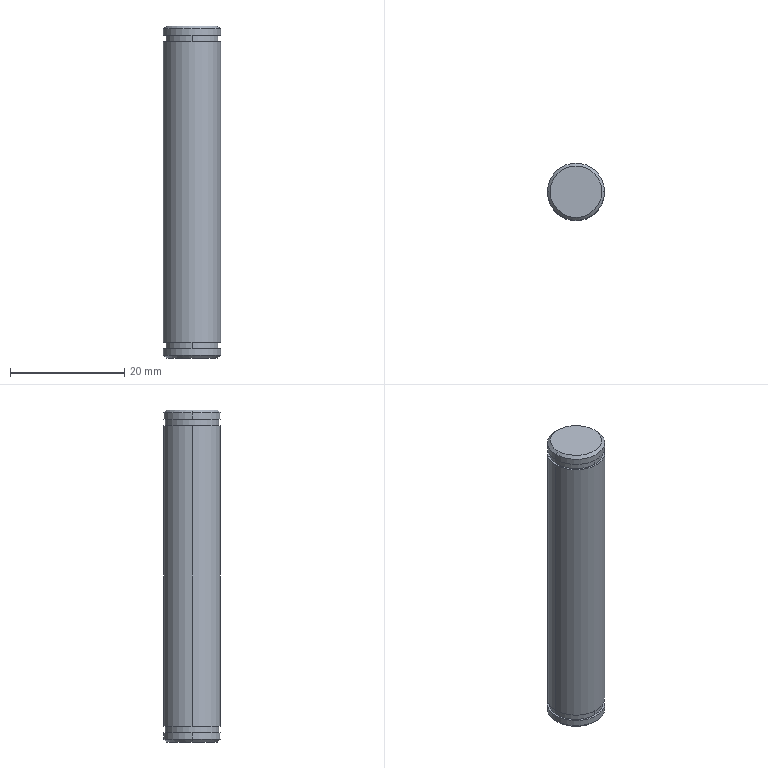Component | SolidWorks | 170423A4-IdlerAssembly5-10_170423A4-IdlerAxis1-1 | 1 solid | 20 faces | box 10 x 10 x 58 mm | volume 4523 mm3 | cylinder 10 | plane 6 | cone 4 | commonest cylinder face diameters 10 x6 9.3 x4
build123d program:
from build123d import *

# Parameters (mm, degrees)
SKETCH1_R           = 5
BOSS_EXTRUDE1_DEPTH = 58
SKETCH2_W           = 1.15
SKETCH2_H           = 0.35
CHAMFER1_SIZE       = 0.5


with BuildPart() as part:
    # Sketch1 → Boss-Extrude1 (new body)
    with BuildSketch(Plane.XY):
        with Locations(Location((0, 0, 0), (0, 0, 180))):
            Circle(SKETCH1_R)
    extrude(amount=BOSS_EXTRUDE1_DEPTH)

    # Sketch2 → Cut-Revolve1 (revolve, cut)
    with BuildSketch(Plane(origin=(0, 0, 0), x_dir=(0, 0, -1), z_dir=(1, 0, 0)), mode=Mode.PRIVATE) as cut_revolve1_sk:
        with Locations((-55.825, 4.825)):
            Rectangle(SKETCH2_W, SKETCH2_H)
        with Locations((-2.175, 4.825)):
            Rectangle(SKETCH2_W, SKETCH2_H)
    revolve(cut_revolve1_sk.sketch.rotate(Axis((0, 0, 58), (0, 0, -1)), 180), axis=Axis((0, 0, 58), (0, 0, -1)), mode=Mode.SUBTRACT)

    # Chamfer1
    chamfer1_edges = [part.edges().sort_by_distance(p)[0] for p in [
        (5, 0, 0),
        (5, 0, 58),
    ]]
    chamfer(chamfer1_edges, length=CHAMFER1_SIZE)


solid = part.part

# Placed as in the assembly
solid = solid.moved(Location((-162.746, 8.712, 412), (0, 0, 0)))
STEP:
#1=COLOUR_RGB('',0.7922,0.8196,0.9333);
#2=FILL_AREA_STYLE_COLOUR('',#1);
#3=FILL_AREA_STYLE('',(#2));
#4=SURFACE_STYLE_FILL_AREA(#3);
#5=SURFACE_SIDE_STYLE('',(#4));
#6=SURFACE_STYLE_USAGE(.BOTH.,#5);
#7=PRESENTATION_STYLE_ASSIGNMENT((#6));
#8=CARTESIAN_POINT('',(-6.585,0.343,18.504));
#9=VERTEX_POINT('',#8);
#10=CARTESIAN_POINT('',(-6.23,0.343,18.504));
#11=VERTEX_POINT('',#10);
#12=CARTESIAN_POINT('',(-6.407,0.343,18.504));
#13=DIRECTION('',(0.,0.,1.));
#14=DIRECTION('',(-1.,0.,0.));
#15=AXIS2_PLACEMENT_3D('',#12,#13,#14);
#16=CIRCLE('',#15,0.1772);
#17=EDGE_CURVE('',#9,#11,#16,.T.);
#18=ORIENTED_EDGE('',*,*,#17,.F.);
#19=CARTESIAN_POINT('',(-6.604,0.343,18.484));
#20=VERTEX_POINT('',#19);
#21=CARTESIAN_POINT('',(-6.585,0.343,18.504));
#22=DIRECTION('',(-0.7071,-0.,-0.7071));
#23=VECTOR('',#22,39.37);
#24=LINE('',#21,#23);
#25=EDGE_CURVE('',#9,#20,#24,.T.);
#26=ORIENTED_EDGE('',*,*,#25,.T.);
#27=CARTESIAN_POINT('',(-6.21,0.343,18.484));
#28=VERTEX_POINT('',#27);
#29=CARTESIAN_POINT('',(-6.407,0.343,18.484));
#30=DIRECTION('',(0.,0.,-1.));
#31=DIRECTION('',(-1.,0.,0.));
#32=AXIS2_PLACEMENT_3D('',#29,#30,#31);
#33=CIRCLE('',#32,0.1969);
#34=EDGE_CURVE('',#28,#20,#33,.T.);
#35=ORIENTED_EDGE('',*,*,#34,.F.);
#36=CARTESIAN_POINT('',(-6.23,0.343,18.504));
#37=DIRECTION('',(0.7071,0.,-0.7071));
#38=VECTOR('',#37,39.37);
#39=LINE('',#36,#38);
#40=EDGE_CURVE('',#11,#28,#39,.T.);
#41=ORIENTED_EDGE('',*,*,#40,.F.);
#42=EDGE_LOOP('',(#18,#26,#35,#41));
#43=FACE_OUTER_BOUND('',#42,.T.);
#44=CARTESIAN_POINT('',(-6.407,0.343,18.504));
#45=DIRECTION('',(0.,0.,-1.));
#46=DIRECTION('',(1.,0.,0.));
#47=AXIS2_PLACEMENT_3D('',#44,#45,#46);
#48=CONICAL_SURFACE('',#47,0.1772,0.7854);
#49=ADVANCED_FACE('',(#43),#48,.T.);
#50=CARTESIAN_POINT('',(-6.23,0.343,16.22));
#51=VERTEX_POINT('',#50);
#52=CARTESIAN_POINT('',(-6.585,0.343,16.22));
#53=VERTEX_POINT('',#52);
#54=CARTESIAN_POINT('',(-6.407,0.343,16.22));
#55=DIRECTION('',(0.,0.,-1.));
#56=DIRECTION('',(-1.,0.,0.));
#57=AXIS2_PLACEMENT_3D('',#54,#55,#56);
#58=CIRCLE('',#57,0.1772);
#59=EDGE_CURVE('',#51,#53,#58,.T.);
#60=ORIENTED_EDGE('',*,*,#59,.F.);
#61=CARTESIAN_POINT('',(-6.21,0.343,16.24));
#62=VERTEX_POINT('',#61);
#63=CARTESIAN_POINT('',(-6.21,0.343,16.24));
#64=DIRECTION('',(0.7071,-0.,0.7071));
#65=VECTOR('',#64,39.37);
#66=LINE('',#63,#65);
#67=EDGE_CURVE('',#51,#62,#66,.T.);
#68=ORIENTED_EDGE('',*,*,#67,.T.);
#69=CARTESIAN_POINT('',(-6.604,0.343,16.24));
#70=VERTEX_POINT('',#69);
#71=CARTESIAN_POINT('',(-6.407,0.343,16.24));
#72=DIRECTION('',(0.,0.,1.));
#73=DIRECTION('',(-1.,0.,0.));
#74=AXIS2_PLACEMENT_3D('',#71,#72,#73);
#75=CIRCLE('',#74,0.1969);
#76=EDGE_CURVE('',#70,#62,#75,.T.);
#77=ORIENTED_EDGE('',*,*,#76,.F.);
#78=CARTESIAN_POINT('',(-6.604,0.343,16.24));
#79=DIRECTION('',(-0.7071,-0.,0.7071));
#80=VECTOR('',#79,39.37);
#81=LINE('',#78,#80);
#82=EDGE_CURVE('',#53,#70,#81,.T.);
#83=ORIENTED_EDGE('',*,*,#82,.F.);
#84=EDGE_LOOP('',(#60,#68,#77,#83));
#85=FACE_OUTER_BOUND('',#84,.T.);
#86=CARTESIAN_POINT('',(-6.407,0.343,16.24));
#87=DIRECTION('',(0.,0.,1.));
#88=DIRECTION('',(-1.,0.,0.));
#89=AXIS2_PLACEMENT_3D('',#86,#87,#88);
#90=CONICAL_SURFACE('',#89,0.1969,0.7854);
#91=ADVANCED_FACE('',(#85),#90,.T.);
#92=CARTESIAN_POINT('',(-6.604,0.343,16.283));
#93=VERTEX_POINT('',#92);
#94=CARTESIAN_POINT('',(-6.21,0.343,16.283));
#95=VERTEX_POINT('',#94);
#96=CARTESIAN_POINT('',(-6.407,0.343,16.283));
#97=DIRECTION('',(-0.,0.,1.));
#98=DIRECTION('',(0.,1.,0.));
#99=AXIS2_PLACEMENT_3D('',#96,#97,#98);
#100=CIRCLE('',#99,0.1969);
#101=EDGE_CURVE('',#93,#95,#100,.T.);
#102=ORIENTED_EDGE('',*,*,#101,.F.);
#103=CARTESIAN_POINT('',(-6.604,0.343,18.504));
#104=DIRECTION('',(0.,0.,-1.));
#105=VECTOR('',#104,39.37);
#106=LINE('',#103,#105);
#107=EDGE_CURVE('',#93,#70,#106,.T.);
#108=ORIENTED_EDGE('',*,*,#107,.T.);
#109=ORIENTED_EDGE('',*,*,#76,.T.);
#110=CARTESIAN_POINT('',(-6.21,0.343,18.504));
#111=DIRECTION('',(0.,0.,-1.));
#112=VECTOR('',#111,39.37);
#113=LINE('',#110,#112);
#114=EDGE_CURVE('',#95,#62,#113,.T.);
#115=ORIENTED_EDGE('',*,*,#114,.F.);
#116=EDGE_LOOP('',(#102,#108,#109,#115));
#117=FACE_OUTER_BOUND('',#116,.T.);
#118=CARTESIAN_POINT('',(-6.407,0.343,18.504));
#119=DIRECTION('',(0.,0.,-1.));
#120=DIRECTION('',(1.,0.,0.));
#121=AXIS2_PLACEMENT_3D('',#118,#119,#120);
#122=CYLINDRICAL_SURFACE('',#121,0.1969);
#123=ADVANCED_FACE('',(#117),#122,.T.);
#124=CARTESIAN_POINT('',(-6.407,0.5261,16.283));
#125=VERTEX_POINT('',#124);
#126=CARTESIAN_POINT('',(-6.407,0.1599,16.283));
#127=VERTEX_POINT('',#126);
#128=CARTESIAN_POINT('',(-6.407,0.343,16.283));
#129=DIRECTION('',(-0.,0.,1.));
#130=DIRECTION('',(0.,1.,0.));
#131=AXIS2_PLACEMENT_3D('',#128,#129,#130);
#132=CIRCLE('',#131,0.1831);
#133=EDGE_CURVE('',#125,#127,#132,.T.);
#134=ORIENTED_EDGE('',*,*,#133,.T.);
#135=CARTESIAN_POINT('',(-6.407,0.1599,16.329));
#136=VERTEX_POINT('',#135);
#137=CARTESIAN_POINT('',(-6.407,0.1599,18.504));
#138=DIRECTION('',(-0.,0.,1.));
#139=VECTOR('',#138,39.37);
#140=LINE('',#137,#139);
#141=EDGE_CURVE('',#127,#136,#140,.T.);
#142=ORIENTED_EDGE('',*,*,#141,.T.);
#143=CARTESIAN_POINT('',(-6.407,0.5261,16.329));
#144=VERTEX_POINT('',#143);
#145=CARTESIAN_POINT('',(-6.407,0.343,16.329));
#146=DIRECTION('',(-0.,0.,1.));
#147=DIRECTION('',(0.,1.,0.));
#148=AXIS2_PLACEMENT_3D('',#145,#146,#147);
#149=CIRCLE('',#148,0.1831);
#150=EDGE_CURVE('',#144,#136,#149,.T.);
#151=ORIENTED_EDGE('',*,*,#150,.F.);
#152=CARTESIAN_POINT('',(-6.407,0.5261,18.504));
#153=DIRECTION('',(-0.,0.,1.));
#154=VECTOR('',#153,39.37);
#155=LINE('',#152,#154);
#156=EDGE_CURVE('',#125,#144,#155,.T.);
#157=ORIENTED_EDGE('',*,*,#156,.F.);
#158=EDGE_LOOP('',(#134,#142,#151,#157));
#159=FACE_OUTER_BOUND('',#158,.T.);
#160=CARTESIAN_POINT('',(-6.407,0.343,18.504));
#161=DIRECTION('',(-0.,0.,1.));
#162=DIRECTION('',(0.,1.,0.));
#163=AXIS2_PLACEMENT_3D('',#160,#161,#162);
#164=CYLINDRICAL_SURFACE('',#163,0.1831);
#165=ADVANCED_FACE('',(#159),#164,.T.);
#166=CARTESIAN_POINT('',(-6.407,0.5261,18.396));
#167=VERTEX_POINT('',#166);
#168=CARTESIAN_POINT('',(-6.407,0.1599,18.396));
#169=VERTEX_POINT('',#168);
#170=CARTESIAN_POINT('',(-6.407,0.343,18.396));
#171=DIRECTION('',(-0.,0.,1.));
#172=DIRECTION('',(0.,1.,0.));
#173=AXIS2_PLACEMENT_3D('',#170,#171,#172);
#174=CIRCLE('',#173,0.1831);
#175=EDGE_CURVE('',#167,#169,#174,.T.);
#176=ORIENTED_EDGE('',*,*,#175,.T.);
#177=CARTESIAN_POINT('',(-6.407,0.1599,18.441));
#178=VERTEX_POINT('',#177);
#179=CARTESIAN_POINT('',(-6.407,0.1599,18.504));
#180=DIRECTION('',(-0.,0.,1.));
#181=VECTOR('',#180,39.37);
#182=LINE('',#179,#181);
#183=EDGE_CURVE('',#169,#178,#182,.T.);
#184=ORIENTED_EDGE('',*,*,#183,.T.);
#185=CARTESIAN_POINT('',(-6.407,0.5261,18.441));
#186=VERTEX_POINT('',#185);
#187=CARTESIAN_POINT('',(-6.407,0.343,18.441));
#188=DIRECTION('',(-0.,0.,1.));
#189=DIRECTION('',(0.,1.,0.));
#190=AXIS2_PLACEMENT_3D('',#187,#188,#189);
#191=CIRCLE('',#190,0.1831);
#192=EDGE_CURVE('',#186,#178,#191,.T.);
#193=ORIENTED_EDGE('',*,*,#192,.F.);
#194=CARTESIAN_POINT('',(-6.407,0.5261,18.504));
#195=DIRECTION('',(-0.,0.,1.));
#196=VECTOR('',#195,39.37);
#197=LINE('',#194,#196);
#198=EDGE_CURVE('',#167,#186,#197,.T.);
#199=ORIENTED_EDGE('',*,*,#198,.F.);
#200=EDGE_LOOP('',(#176,#184,#193,#199));
#201=FACE_OUTER_BOUND('',#200,.T.);
#202=CARTESIAN_POINT('',(-6.407,0.343,18.504));
#203=DIRECTION('',(-0.,0.,1.));
#204=DIRECTION('',(0.,1.,0.));
#205=AXIS2_PLACEMENT_3D('',#202,#203,#204);
#206=CYLINDRICAL_SURFACE('',#205,0.1831);
#207=ADVANCED_FACE('',(#201),#206,.T.);
#208=ORIENTED_EDGE('',*,*,#34,.T.);
#209=CARTESIAN_POINT('',(-6.604,0.343,18.441));
#210=VERTEX_POINT('',#209);
#211=CARTESIAN_POINT('',(-6.604,0.343,18.504));
#212=DIRECTION('',(0.,0.,-1.));
#213=VECTOR('',#212,39.37);
#214=LINE('',#211,#213);
#215=EDGE_CURVE('',#20,#210,#214,.T.);
#216=ORIENTED_EDGE('',*,*,#215,.T.);
#217=CARTESIAN_POINT('',(-6.21,0.343,18.441));
#218=VERTEX_POINT('',#217);
#219=CARTESIAN_POINT('',(-6.407,0.343,18.441));
#220=DIRECTION('',(-0.,0.,1.));
#221=DIRECTION('',(0.,1.,0.));
#222=AXIS2_PLACEMENT_3D('',#219,#220,#221);
#223=CIRCLE('',#222,0.1969);
#224=EDGE_CURVE('',#210,#218,#223,.T.);
#225=ORIENTED_EDGE('',*,*,#224,.T.);
#226=CARTESIAN_POINT('',(-6.21,0.343,18.504));
#227=DIRECTION('',(0.,0.,-1.));
#228=VECTOR('',#227,39.37);
#229=LINE('',#226,#228);
#230=EDGE_CURVE('',#28,#218,#229,.T.);
#231=ORIENTED_EDGE('',*,*,#230,.F.);
#232=EDGE_LOOP('',(#208,#216,#225,#231));
#233=FACE_OUTER_BOUND('',#232,.T.);
#234=CARTESIAN_POINT('',(-6.407,0.343,18.504));
#235=DIRECTION('',(0.,0.,-1.));
#236=DIRECTION('',(1.,0.,0.));
#237=AXIS2_PLACEMENT_3D('',#234,#235,#236);
#238=CYLINDRICAL_SURFACE('',#237,0.1969);
#239=ADVANCED_FACE('',(#233),#238,.T.);
#240=CARTESIAN_POINT('',(-6.604,0.343,18.396));
#241=VERTEX_POINT('',#240);
#242=CARTESIAN_POINT('',(-6.21,0.343,18.396));
#243=VERTEX_POINT('',#242);
#244=CARTESIAN_POINT('',(-6.407,0.343,18.396));
#245=DIRECTION('',(-0.,0.,1.));
#246=DIRECTION('',(0.,1.,0.));
#247=AXIS2_PLACEMENT_3D('',#244,#245,#246);
#248=CIRCLE('',#247,0.1969);
#249=EDGE_CURVE('',#241,#243,#248,.T.);
#250=ORIENTED_EDGE('',*,*,#249,.F.);
#251=CARTESIAN_POINT('',(-6.604,0.343,16.329));
#252=VERTEX_POINT('',#251);
#253=CARTESIAN_POINT('',(-6.604,0.343,18.504));
#254=DIRECTION('',(0.,0.,-1.));
#255=VECTOR('',#254,39.37);
#256=LINE('',#253,#255);
#257=EDGE_CURVE('',#241,#252,#256,.T.);
#258=ORIENTED_EDGE('',*,*,#257,.T.);
#259=CARTESIAN_POINT('',(-6.21,0.343,16.329));
#260=VERTEX_POINT('',#259);
#261=CARTESIAN_POINT('',(-6.407,0.343,16.329));
#262=DIRECTION('',(-0.,0.,1.));
#263=DIRECTION('',(0.,1.,0.));
#264=AXIS2_PLACEMENT_3D('',#261,#262,#263);
#265=CIRCLE('',#264,0.1969);
#266=EDGE_CURVE('',#252,#260,#265,.T.);
#267=ORIENTED_EDGE('',*,*,#266,.T.);
#268=CARTESIAN_POINT('',(-6.21,0.343,18.504));
#269=DIRECTION('',(0.,0.,-1.));
#270=VECTOR('',#269,39.37);
#271=LINE('',#268,#270);
#272=EDGE_CURVE('',#243,#260,#271,.T.);
#273=ORIENTED_EDGE('',*,*,#272,.F.);
#274=EDGE_LOOP('',(#250,#258,#267,#273));
#275=FACE_OUTER_BOUND('',#274,.T.);
#276=CARTESIAN_POINT('',(-6.407,0.343,18.504));
#277=DIRECTION('',(0.,0.,-1.));
#278=DIRECTION('',(1.,0.,0.));
#279=AXIS2_PLACEMENT_3D('',#276,#277,#278);
#280=CYLINDRICAL_SURFACE('',#279,0.1969);
#281=ADVANCED_FACE('',(#275),#280,.T.);
#282=ORIENTED_EDGE('',*,*,#257,.F.);
#283=CARTESIAN_POINT('',(-6.407,0.343,18.396));
#284=DIRECTION('',(-0.,0.,1.));
#285=DIRECTION('',(0.,1.,0.));
#286=AXIS2_PLACEMENT_3D('',#283,#284,#285);
#287=CIRCLE('',#286,0.1969);
#288=EDGE_CURVE('',#243,#241,#287,.T.);
#289=ORIENTED_EDGE('',*,*,#288,.F.);
#290=ORIENTED_EDGE('',*,*,#272,.T.);
#291=CARTESIAN_POINT('',(-6.407,0.343,16.329));
#292=DIRECTION('',(-0.,0.,1.));
#293=DIRECTION('',(0.,1.,0.));
#294=AXIS2_PLACEMENT_3D('',#291,#292,#293);
#295=CIRCLE('',#294,0.1969);
#296=EDGE_CURVE('',#260,#252,#295,.T.);
#297=ORIENTED_EDGE('',*,*,#296,.T.);
#298=EDGE_LOOP('',(#282,#289,#290,#297));
#299=FACE_OUTER_BOUND('',#298,.T.);
#300=CARTESIAN_POINT('',(-6.407,0.343,18.504));
#301=DIRECTION('',(0.,0.,-1.));
#302=DIRECTION('',(1.,0.,0.));
#303=AXIS2_PLACEMENT_3D('',#300,#301,#302);
#304=CYLINDRICAL_SURFACE('',#303,0.1969);
#305=ADVANCED_FACE('',(#299),#304,.T.);
#306=ORIENTED_EDGE('',*,*,#215,.F.);
#307=CARTESIAN_POINT('',(-6.407,0.343,18.484));
#308=DIRECTION('',(0.,0.,-1.));
#309=DIRECTION('',(-1.,0.,0.));
#310=AXIS2_PLACEMENT_3D('',#307,#308,#309);
#311=CIRCLE('',#310,0.1969);
#312=EDGE_CURVE('',#20,#28,#311,.T.);
#313=ORIENTED_EDGE('',*,*,#312,.T.);
#314=ORIENTED_EDGE('',*,*,#230,.T.);
#315=CARTESIAN_POINT('',(-6.407,0.343,18.441));
#316=DIRECTION('',(-0.,0.,1.));
#317=DIRECTION('',(0.,1.,0.));
#318=AXIS2_PLACEMENT_3D('',#315,#316,#317);
#319=CIRCLE('',#318,0.1969);
#320=EDGE_CURVE('',#218,#210,#319,.T.);
#321=ORIENTED_EDGE('',*,*,#320,.T.);
#322=EDGE_LOOP('',(#306,#313,#314,#321));
#323=FACE_OUTER_BOUND('',#322,.T.);
#324=CARTESIAN_POINT('',(-6.407,0.343,18.504));
#325=DIRECTION('',(0.,0.,-1.));
#326=DIRECTION('',(1.,0.,0.));
#327=AXIS2_PLACEMENT_3D('',#324,#325,#326);
#328=CYLINDRICAL_SURFACE('',#327,0.1969);
#329=ADVANCED_FACE('',(#323),#328,.T.);
#330=CARTESIAN_POINT('',(-6.407,0.343,18.504));
#331=DIRECTION('',(0.,0.,1.));
#332=DIRECTION('',(-1.,0.,0.));
#333=AXIS2_PLACEMENT_3D('',#330,#331,#332);
#334=CIRCLE('',#333,0.1772);
#335=EDGE_CURVE('',#11,#9,#334,.T.);
#336=ORIENTED_EDGE('',*,*,#335,.T.);
#337=ORIENTED_EDGE('',*,*,#17,.T.);
#338=EDGE_LOOP('',(#336,#337));
#339=FACE_OUTER_BOUND('',#338,.T.);
#340=CARTESIAN_POINT('',(-6.407,0.343,18.504));
#341=DIRECTION('',(0.,0.,1.));
#342=DIRECTION('',(-1.,-0.,0.));
#343=AXIS2_PLACEMENT_3D('',#340,#341,#342);
#344=PLANE('',#343);
#345=ADVANCED_FACE('',(#339),#344,.T.);
#346=ORIENTED_EDGE('',*,*,#192,.T.);
#347=CARTESIAN_POINT('',(-6.407,0.343,18.441));
#348=DIRECTION('',(-0.,0.,1.));
#349=DIRECTION('',(0.,1.,0.));
#350=AXIS2_PLACEMENT_3D('',#347,#348,#349);
#351=CIRCLE('',#350,0.1831);
#352=EDGE_CURVE('',#178,#186,#351,.T.);
#353=ORIENTED_EDGE('',*,*,#352,.T.);
#354=EDGE_LOOP('',(#346,#353));
#355=FACE_BOUND('',#354,.T.);
#356=ORIENTED_EDGE('',*,*,#320,.F.);
#357=ORIENTED_EDGE('',*,*,#224,.F.);
#358=EDGE_LOOP('',(#356,#357));
#359=FACE_OUTER_BOUND('',#358,.T.);
#360=CARTESIAN_POINT('',(-6.407,0.1461,18.441));
#361=DIRECTION('',(0.,-0.,-1.));
#362=DIRECTION('',(0.,-1.,0.));
#363=AXIS2_PLACEMENT_3D('',#360,#361,#362);
#364=PLANE('',#363);
#365=ADVANCED_FACE('',(#355,#359),#364,.T.);
#366=ORIENTED_EDGE('',*,*,#183,.F.);
#367=CARTESIAN_POINT('',(-6.407,0.343,18.396));
#368=DIRECTION('',(-0.,0.,1.));
#369=DIRECTION('',(0.,1.,0.));
#370=AXIS2_PLACEMENT_3D('',#367,#368,#369);
#371=CIRCLE('',#370,0.1831);
#372=EDGE_CURVE('',#169,#167,#371,.T.);
#373=ORIENTED_EDGE('',*,*,#372,.T.);
#374=ORIENTED_EDGE('',*,*,#198,.T.);
#375=ORIENTED_EDGE('',*,*,#352,.F.);
#376=EDGE_LOOP('',(#366,#373,#374,#375));
#377=FACE_OUTER_BOUND('',#376,.T.);
#378=CARTESIAN_POINT('',(-6.407,0.343,18.504));
#379=DIRECTION('',(-0.,0.,1.));
#380=DIRECTION('',(0.,1.,0.));
#381=AXIS2_PLACEMENT_3D('',#378,#379,#380);
#382=CYLINDRICAL_SURFACE('',#381,0.1831);
#383=ADVANCED_FACE('',(#377),#382,.T.);
#384=ORIENTED_EDGE('',*,*,#288,.T.);
#385=ORIENTED_EDGE('',*,*,#249,.T.);
#386=EDGE_LOOP('',(#384,#385));
#387=FACE_OUTER_BOUND('',#386,.T.);
#388=ORIENTED_EDGE('',*,*,#175,.F.);
#389=ORIENTED_EDGE('',*,*,#372,.F.);
#390=EDGE_LOOP('',(#388,#389));
#391=FACE_BOUND('',#390,.T.);
#392=CARTESIAN_POINT('',(-6.407,0.1461,18.396));
#393=DIRECTION('',(-0.,0.,1.));
#394=DIRECTION('',(-0.,1.,-0.));
#395=AXIS2_PLACEMENT_3D('',#392,#393,#394);
#396=PLANE('',#395);
#397=ADVANCED_FACE('',(#387,#391),#396,.T.);
#398=ORIENTED_EDGE('',*,*,#150,.T.);
#399=CARTESIAN_POINT('',(-6.407,0.343,16.329));
#400=DIRECTION('',(-0.,0.,1.));
#401=DIRECTION('',(0.,1.,0.));
#402=AXIS2_PLACEMENT_3D('',#399,#400,#401);
#403=CIRCLE('',#402,0.1831);
#404=EDGE_CURVE('',#136,#144,#403,.T.);
#405=ORIENTED_EDGE('',*,*,#404,.T.);
#406=EDGE_LOOP('',(#398,#405));
#407=FACE_BOUND('',#406,.T.);
#408=ORIENTED_EDGE('',*,*,#296,.F.);
#409=ORIENTED_EDGE('',*,*,#266,.F.);
#410=EDGE_LOOP('',(#408,#409));
#411=FACE_OUTER_BOUND('',#410,.T.);
#412=CARTESIAN_POINT('',(-6.407,0.1461,16.329));
#413=DIRECTION('',(0.,-0.,-1.));
#414=DIRECTION('',(0.,-1.,0.));
#415=AXIS2_PLACEMENT_3D('',#412,#413,#414);
#416=PLANE('',#415);
#417=ADVANCED_FACE('',(#407,#411),#416,.T.);
#418=ORIENTED_EDGE('',*,*,#141,.F.);
#419=CARTESIAN_POINT('',(-6.407,0.343,16.283));
#420=DIRECTION('',(-0.,0.,1.));
#421=DIRECTION('',(0.,1.,0.));
#422=AXIS2_PLACEMENT_3D('',#419,#420,#421);
#423=CIRCLE('',#422,0.1831);
#424=EDGE_CURVE('',#127,#125,#423,.T.);
#425=ORIENTED_EDGE('',*,*,#424,.T.);
#426=ORIENTED_EDGE('',*,*,#156,.T.);
#427=ORIENTED_EDGE('',*,*,#404,.F.);
#428=EDGE_LOOP('',(#418,#425,#426,#427));
#429=FACE_OUTER_BOUND('',#428,.T.);
#430=CARTESIAN_POINT('',(-6.407,0.343,18.504));
#431=DIRECTION('',(-0.,0.,1.));
#432=DIRECTION('',(0.,1.,0.));
#433=AXIS2_PLACEMENT_3D('',#430,#431,#432);
#434=CYLINDRICAL_SURFACE('',#433,0.1831);
#435=ADVANCED_FACE('',(#429),#434,.T.);
#436=CARTESIAN_POINT('',(-6.407,0.343,16.283));
#437=DIRECTION('',(-0.,0.,1.));
#438=DIRECTION('',(0.,1.,0.));
#439=AXIS2_PLACEMENT_3D('',#436,#437,#438);
#440=CIRCLE('',#439,0.1969);
#441=EDGE_CURVE('',#95,#93,#440,.T.);
#442=ORIENTED_EDGE('',*,*,#441,.T.);
#443=ORIENTED_EDGE('',*,*,#101,.T.);
#444=EDGE_LOOP('',(#442,#443));
#445=FACE_OUTER_BOUND('',#444,.T.);
#446=ORIENTED_EDGE('',*,*,#133,.F.);
#447=ORIENTED_EDGE('',*,*,#424,.F.);
#448=EDGE_LOOP('',(#446,#447));
#449=FACE_BOUND('',#448,.T.);
#450=CARTESIAN_POINT('',(-6.407,0.1461,16.283));
#451=DIRECTION('',(-0.,0.,1.));
#452=DIRECTION('',(-0.,1.,-0.));
#453=AXIS2_PLACEMENT_3D('',#450,#451,#452);
#454=PLANE('',#453);
#455=ADVANCED_FACE('',(#445,#449),#454,.T.);
#456=CARTESIAN_POINT('',(-6.407,0.343,16.22));
#457=DIRECTION('',(0.,0.,-1.));
#458=DIRECTION('',(-1.,0.,0.));
#459=AXIS2_PLACEMENT_3D('',#456,#457,#458);
#460=CIRCLE('',#459,0.1772);
#461=EDGE_CURVE('',#53,#51,#460,.T.);
#462=ORIENTED_EDGE('',*,*,#461,.T.);
#463=ORIENTED_EDGE('',*,*,#59,.T.);
#464=EDGE_LOOP('',(#462,#463));
#465=FACE_OUTER_BOUND('',#464,.T.);
#466=CARTESIAN_POINT('',(-6.407,0.343,16.22));
#467=DIRECTION('',(0.,0.,1.));
#468=DIRECTION('',(-1.,-0.,0.));
#469=AXIS2_PLACEMENT_3D('',#466,#467,#468);
#470=PLANE('',#469);
#471=ADVANCED_FACE('',(#465),#470,.F.);
#472=ORIENTED_EDGE('',*,*,#107,.F.);
#473=ORIENTED_EDGE('',*,*,#441,.F.);
#474=ORIENTED_EDGE('',*,*,#114,.T.);
#475=CARTESIAN_POINT('',(-6.407,0.343,16.24));
#476=DIRECTION('',(0.,0.,1.));
#477=DIRECTION('',(-1.,0.,0.));
#478=AXIS2_PLACEMENT_3D('',#475,#476,#477);
#479=CIRCLE('',#478,0.1969);
#480=EDGE_CURVE('',#62,#70,#479,.T.);
#481=ORIENTED_EDGE('',*,*,#480,.T.);
#482=EDGE_LOOP('',(#472,#473,#474,#481));
#483=FACE_OUTER_BOUND('',#482,.T.);
#484=CARTESIAN_POINT('',(-6.407,0.343,18.504));
#485=DIRECTION('',(0.,0.,-1.));
#486=DIRECTION('',(1.,0.,0.));
#487=AXIS2_PLACEMENT_3D('',#484,#485,#486);
#488=CYLINDRICAL_SURFACE('',#487,0.1969);
#489=ADVANCED_FACE('',(#483),#488,.T.);
#490=ORIENTED_EDGE('',*,*,#67,.F.);
#491=ORIENTED_EDGE('',*,*,#461,.F.);
#492=ORIENTED_EDGE('',*,*,#82,.T.);
#493=ORIENTED_EDGE('',*,*,#480,.F.);
#494=EDGE_LOOP('',(#490,#491,#492,#493));
#495=FACE_OUTER_BOUND('',#494,.T.);
#496=CARTESIAN_POINT('',(-6.407,0.343,16.24));
#497=DIRECTION('',(0.,0.,1.));
#498=DIRECTION('',(-1.,0.,0.));
#499=AXIS2_PLACEMENT_3D('',#496,#497,#498);
#500=CONICAL_SURFACE('',#499,0.1969,0.7854);
#501=ADVANCED_FACE('',(#495),#500,.T.);
#502=ORIENTED_EDGE('',*,*,#25,.F.);
#503=ORIENTED_EDGE('',*,*,#335,.F.);
#504=ORIENTED_EDGE('',*,*,#40,.T.);
#505=ORIENTED_EDGE('',*,*,#312,.F.);
#506=EDGE_LOOP('',(#502,#503,#504,#505));
#507=FACE_OUTER_BOUND('',#506,.T.);
#508=CARTESIAN_POINT('',(-6.407,0.343,18.504));
#509=DIRECTION('',(0.,0.,-1.));
#510=DIRECTION('',(1.,0.,0.));
#511=AXIS2_PLACEMENT_3D('',#508,#509,#510);
#512=CONICAL_SURFACE('',#511,0.1772,0.7854);
#513=ADVANCED_FACE('',(#507),#512,.T.);
#514=CLOSED_SHELL('',(#49,#91,#123,#165,#207,#239,#281,#305,#329,#345,#365,#383,#397,#417,#435,#455,#471,#489,#501,#513));
#515=MANIFOLD_SOLID_BREP('',#514);
#516=STYLED_ITEM('',(#7),#515);
#517=(LENGTH_UNIT()NAMED_UNIT(*)SI_UNIT($,.METRE.));
#518=LENGTH_MEASURE_WITH_UNIT(LENGTH_MEASURE(0.0254),#517);
#519=DIMENSIONAL_EXPONENTS(1.,0.,0.,0.,0.,0.,0.);
#520=(CONVERSION_BASED_UNIT('',#518)LENGTH_UNIT()NAMED_UNIT(#519));
#521=UNCERTAINTY_MEASURE_WITH_UNIT(LENGTH_MEASURE(0.00001),#520,'','');
#522=(NAMED_UNIT(*)PLANE_ANGLE_UNIT()SI_UNIT($,.RADIAN.));
#523=(NAMED_UNIT(*)SI_UNIT($,.STERADIAN.)SOLID_ANGLE_UNIT());
#524=(GEOMETRIC_REPRESENTATION_CONTEXT(3)GLOBAL_UNCERTAINTY_ASSIGNED_CONTEXT((#521))GLOBAL_UNIT_ASSIGNED_CONTEXT((#520,#522,#523))REPRESENTATION_CONTEXT('',''));
#525=MECHANICAL_DESIGN_GEOMETRIC_PRESENTATION_REPRESENTATION('',(#516),#524);
#526=PRESENTATION_LAYER_ASSIGNMENT('','',(#516));
#527=CARTESIAN_POINT('',(0.,0.,0.));
#528=DIRECTION('',(0.,0.,1.));
#529=DIRECTION('',(1.,0.,0.));
#530=AXIS2_PLACEMENT_3D('',#527,#528,#529);
#531=(LENGTH_UNIT()NAMED_UNIT(*)SI_UNIT($,.METRE.));
#532=LENGTH_MEASURE_WITH_UNIT(LENGTH_MEASURE(0.0254),#531);
#533=DIMENSIONAL_EXPONENTS(1.,0.,0.,0.,0.,0.,0.);
#534=(CONVERSION_BASED_UNIT('',#532)LENGTH_UNIT()NAMED_UNIT(#533));
#535=UNCERTAINTY_MEASURE_WITH_UNIT(LENGTH_MEASURE(0.00001),#534,'','');
#536=(NAMED_UNIT(*)PLANE_ANGLE_UNIT()SI_UNIT($,.RADIAN.));
#537=(NAMED_UNIT(*)SI_UNIT($,.STERADIAN.)SOLID_ANGLE_UNIT());
#538=(GEOMETRIC_REPRESENTATION_CONTEXT(3)GLOBAL_UNCERTAINTY_ASSIGNED_CONTEXT((#535))GLOBAL_UNIT_ASSIGNED_CONTEXT((#534,#536,#537))REPRESENTATION_CONTEXT('',''));
#539=ADVANCED_BREP_SHAPE_REPRESENTATION('',(#515,#530),#538);